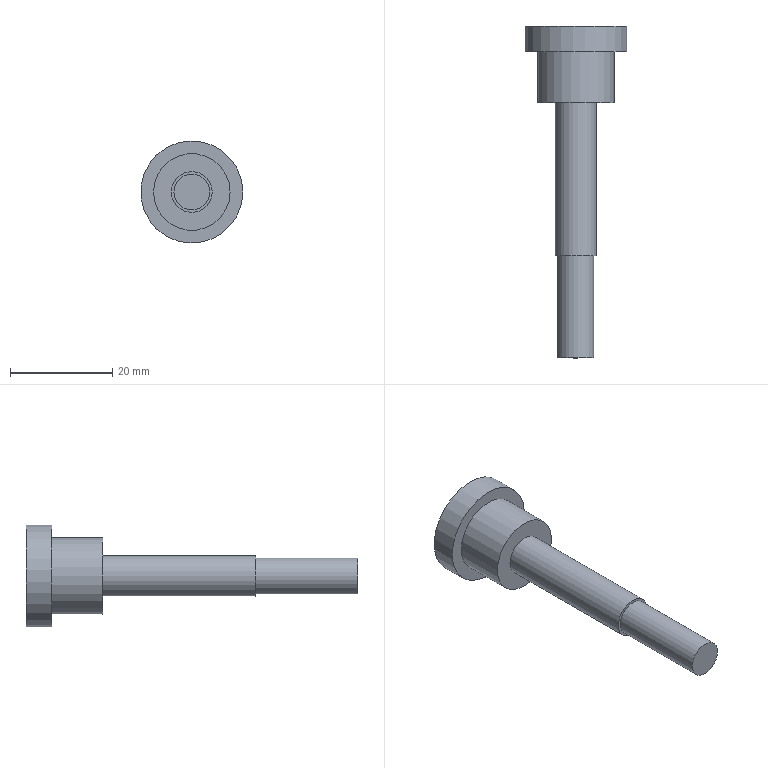Component | NX | HANDLE | 1 solid | 9 faces | box 20 x 65 x 20 mm | volume 5616 mm3 | plane 5 | cylinder 4 | commonest cylinder face diameters 7 x1 8 x1 15 x1 20 x1
STEP:
#1=CARTESIAN_POINT('',(0.,0.,0.));
#2=DIRECTION('',(0.,0.,1.));
#3=DIRECTION('',(1.,0.,0.));
#4=AXIS2_PLACEMENT_3D('',#1,#2,#3);
#5=CARTESIAN_POINT('',(28.011,213.604,30.));
#6=VERTEX_POINT('',#5);
#7=CARTESIAN_POINT('',(24.511,213.604,30.));
#8=DIRECTION('',(0.,1.,0.));
#9=DIRECTION('',(1.,0.,0.));
#10=AXIS2_PLACEMENT_3D('',#7,#8,#9);
#11=CIRCLE('',#10,3.5);
#12=CARTESIAN_POINT('',(24.511,213.604,30.));
#13=DIRECTION('',(0.,-1.,0.));
#14=DIRECTION('',(-1.,0.,0.));
#15=AXIS2_PLACEMENT_3D('',#12,#13,#14);
#16=CYLINDRICAL_SURFACE('',#15,3.5);
#17=CARTESIAN_POINT('',(9.425,0.));
#18=DIRECTION('',(-1.,0.));
#19=VECTOR('',#18,1.);
#20=LINE('',#17,#19);
#21=(GEOMETRIC_REPRESENTATION_CONTEXT(2)PARAMETRIC_REPRESENTATION_CONTEXT()REPRESENTATION_CONTEXT('',''));
#22=DEFINITIONAL_REPRESENTATION('',(#20),#21);
#23=PCURVE('',#16,#22);
#24=CARTESIAN_POINT('',(24.511,213.604,30.));
#25=DIRECTION('',(0.,1.,0.));
#26=DIRECTION('',(1.,0.,0.));
#27=AXIS2_PLACEMENT_3D('',#24,#25,#26);
#28=PLANE('',#27);
#29=CARTESIAN_POINT('',(0.,0.));
#30=DIRECTION('',(1.,0.));
#31=AXIS2_PLACEMENT_2D('',#29,#30);
#32=CIRCLE('',#31,3.5);
#33=(GEOMETRIC_REPRESENTATION_CONTEXT(2)PARAMETRIC_REPRESENTATION_CONTEXT()REPRESENTATION_CONTEXT('',''));
#34=DEFINITIONAL_REPRESENTATION('',(#32),#33);
#35=PCURVE('',#28,#34);
#36=SURFACE_CURVE('',#11,(#23,#35),.PCURVE_S1.);
#37=EDGE_CURVE('',#6,#6,#36,.T.);
#38=ORIENTED_EDGE('',*,*,#37,.F.);
#39=CARTESIAN_POINT('',(28.011,193.604,30.));
#40=VERTEX_POINT('',#39);
#41=CARTESIAN_POINT('',(28.011,213.604,30.));
#42=CARTESIAN_POINT('',(28.011,193.604,30.));
#43=B_SPLINE_CURVE_WITH_KNOTS('',1,(#41,#42),.UNSPECIFIED.,.F.,.F.,(2,2),(0.,20.),.PIECEWISE_BEZIER_KNOTS.);
#44=CARTESIAN_POINT('',(9.425,0.));
#45=DIRECTION('',(0.,1.));
#46=VECTOR('',#45,1.);
#47=LINE('',#44,#46);
#48=(GEOMETRIC_REPRESENTATION_CONTEXT(2)PARAMETRIC_REPRESENTATION_CONTEXT()REPRESENTATION_CONTEXT('',''));
#49=DEFINITIONAL_REPRESENTATION('',(#47),#48);
#50=PCURVE('',#16,#49);
#51=CARTESIAN_POINT('',(3.142,0.));
#52=DIRECTION('',(0.,1.));
#53=VECTOR('',#52,1.);
#54=LINE('',#51,#53);
#55=(GEOMETRIC_REPRESENTATION_CONTEXT(2)PARAMETRIC_REPRESENTATION_CONTEXT()REPRESENTATION_CONTEXT('',''));
#56=DEFINITIONAL_REPRESENTATION('',(#54),#55);
#57=PCURVE('',#16,#56);
#58=SEAM_CURVE('',#43,(#50,#57),.PCURVE_S1.);
#59=EDGE_CURVE('',#6,#40,#58,.T.);
#60=ORIENTED_EDGE('',*,*,#59,.T.);
#61=CARTESIAN_POINT('',(24.511,193.604,30.));
#62=DIRECTION('',(0.,1.,0.));
#63=DIRECTION('',(1.,0.,0.));
#64=AXIS2_PLACEMENT_3D('',#61,#62,#63);
#65=CIRCLE('',#64,3.5);
#66=CARTESIAN_POINT('',(9.425,20.));
#67=DIRECTION('',(-1.,0.));
#68=VECTOR('',#67,1.);
#69=LINE('',#66,#68);
#70=(GEOMETRIC_REPRESENTATION_CONTEXT(2)PARAMETRIC_REPRESENTATION_CONTEXT()REPRESENTATION_CONTEXT('',''));
#71=DEFINITIONAL_REPRESENTATION('',(#69),#70);
#72=PCURVE('',#16,#71);
#73=CARTESIAN_POINT('',(24.511,193.604,30.));
#74=DIRECTION('',(0.,1.,0.));
#75=DIRECTION('',(1.,0.,0.));
#76=AXIS2_PLACEMENT_3D('',#73,#74,#75);
#77=PLANE('',#76);
#78=CARTESIAN_POINT('',(0.,0.));
#79=DIRECTION('',(1.,0.));
#80=AXIS2_PLACEMENT_2D('',#78,#79);
#81=CIRCLE('',#80,3.5);
#82=(GEOMETRIC_REPRESENTATION_CONTEXT(2)PARAMETRIC_REPRESENTATION_CONTEXT()REPRESENTATION_CONTEXT('',''));
#83=DEFINITIONAL_REPRESENTATION('',(#81),#82);
#84=PCURVE('',#77,#83);
#85=SURFACE_CURVE('',#65,(#72,#84),.PCURVE_S1.);
#86=EDGE_CURVE('',#40,#40,#85,.T.);
#87=ORIENTED_EDGE('',*,*,#86,.T.);
#88=ORIENTED_EDGE('',*,*,#59,.F.);
#89=EDGE_LOOP('',(#38,#60,#87,#88));
#90=FACE_BOUND('',#89,.T.);
#91=ADVANCED_FACE('',(#90),#16,.T.);
#92=ORIENTED_EDGE('',*,*,#86,.F.);
#93=EDGE_LOOP('',(#92));
#94=FACE_BOUND('',#93,.T.);
#95=ADVANCED_FACE('',(#94),#77,.F.);
#96=CARTESIAN_POINT('',(28.511,243.604,30.));
#97=VERTEX_POINT('',#96);
#98=CARTESIAN_POINT('',(24.511,243.604,30.));
#99=DIRECTION('',(0.,1.,0.));
#100=DIRECTION('',(1.,0.,0.));
#101=AXIS2_PLACEMENT_3D('',#98,#99,#100);
#102=CIRCLE('',#101,4.);
#103=CARTESIAN_POINT('',(24.511,243.604,30.));
#104=DIRECTION('',(0.,-1.,0.));
#105=DIRECTION('',(-1.,0.,0.));
#106=AXIS2_PLACEMENT_3D('',#103,#104,#105);
#107=CYLINDRICAL_SURFACE('',#106,4.);
#108=CARTESIAN_POINT('',(9.425,0.));
#109=DIRECTION('',(-1.,0.));
#110=VECTOR('',#109,1.);
#111=LINE('',#108,#110);
#112=(GEOMETRIC_REPRESENTATION_CONTEXT(2)PARAMETRIC_REPRESENTATION_CONTEXT()REPRESENTATION_CONTEXT('',''));
#113=DEFINITIONAL_REPRESENTATION('',(#111),#112);
#114=PCURVE('',#107,#113);
#115=CARTESIAN_POINT('',(24.511,243.604,30.));
#116=DIRECTION('',(0.,1.,0.));
#117=DIRECTION('',(1.,0.,0.));
#118=AXIS2_PLACEMENT_3D('',#115,#116,#117);
#119=PLANE('',#118);
#120=CARTESIAN_POINT('',(0.,0.));
#121=DIRECTION('',(1.,0.));
#122=AXIS2_PLACEMENT_2D('',#120,#121);
#123=CIRCLE('',#122,4.);
#124=(GEOMETRIC_REPRESENTATION_CONTEXT(2)PARAMETRIC_REPRESENTATION_CONTEXT()REPRESENTATION_CONTEXT('',''));
#125=DEFINITIONAL_REPRESENTATION('',(#123),#124);
#126=PCURVE('',#119,#125);
#127=SURFACE_CURVE('',#102,(#114,#126),.PCURVE_S1.);
#128=EDGE_CURVE('',#97,#97,#127,.T.);
#129=ORIENTED_EDGE('',*,*,#128,.F.);
#130=CARTESIAN_POINT('',(28.511,213.604,30.));
#131=VERTEX_POINT('',#130);
#132=CARTESIAN_POINT('',(28.511,243.604,30.));
#133=CARTESIAN_POINT('',(28.511,213.604,30.));
#134=B_SPLINE_CURVE_WITH_KNOTS('',1,(#132,#133),.UNSPECIFIED.,.F.,.F.,(2,2),(0.,30.),.PIECEWISE_BEZIER_KNOTS.);
#135=CARTESIAN_POINT('',(9.425,0.));
#136=DIRECTION('',(0.,1.));
#137=VECTOR('',#136,1.);
#138=LINE('',#135,#137);
#139=(GEOMETRIC_REPRESENTATION_CONTEXT(2)PARAMETRIC_REPRESENTATION_CONTEXT()REPRESENTATION_CONTEXT('',''));
#140=DEFINITIONAL_REPRESENTATION('',(#138),#139);
#141=PCURVE('',#107,#140);
#142=CARTESIAN_POINT('',(3.142,0.));
#143=DIRECTION('',(0.,1.));
#144=VECTOR('',#143,1.);
#145=LINE('',#142,#144);
#146=(GEOMETRIC_REPRESENTATION_CONTEXT(2)PARAMETRIC_REPRESENTATION_CONTEXT()REPRESENTATION_CONTEXT('',''));
#147=DEFINITIONAL_REPRESENTATION('',(#145),#146);
#148=PCURVE('',#107,#147);
#149=SEAM_CURVE('',#134,(#141,#148),.PCURVE_S1.);
#150=EDGE_CURVE('',#97,#131,#149,.T.);
#151=ORIENTED_EDGE('',*,*,#150,.T.);
#152=CARTESIAN_POINT('',(24.511,213.604,30.));
#153=DIRECTION('',(0.,1.,0.));
#154=DIRECTION('',(1.,0.,0.));
#155=AXIS2_PLACEMENT_3D('',#152,#153,#154);
#156=CIRCLE('',#155,4.);
#157=CARTESIAN_POINT('',(9.425,30.));
#158=DIRECTION('',(-1.,0.));
#159=VECTOR('',#158,1.);
#160=LINE('',#157,#159);
#161=(GEOMETRIC_REPRESENTATION_CONTEXT(2)PARAMETRIC_REPRESENTATION_CONTEXT()REPRESENTATION_CONTEXT('',''));
#162=DEFINITIONAL_REPRESENTATION('',(#160),#161);
#163=PCURVE('',#107,#162);
#164=CARTESIAN_POINT('',(0.,0.));
#165=DIRECTION('',(1.,0.));
#166=AXIS2_PLACEMENT_2D('',#164,#165);
#167=CIRCLE('',#166,4.);
#168=(GEOMETRIC_REPRESENTATION_CONTEXT(2)PARAMETRIC_REPRESENTATION_CONTEXT()REPRESENTATION_CONTEXT('',''));
#169=DEFINITIONAL_REPRESENTATION('',(#167),#168);
#170=PCURVE('',#28,#169);
#171=SURFACE_CURVE('',#156,(#163,#170),.PCURVE_S1.);
#172=EDGE_CURVE('',#131,#131,#171,.T.);
#173=ORIENTED_EDGE('',*,*,#172,.T.);
#174=ORIENTED_EDGE('',*,*,#150,.F.);
#175=EDGE_LOOP('',(#129,#151,#173,#174));
#176=FACE_BOUND('',#175,.T.);
#177=ADVANCED_FACE('',(#176),#107,.T.);
#178=ORIENTED_EDGE('',*,*,#37,.T.);
#179=EDGE_LOOP('',(#178));
#180=FACE_BOUND('',#179,.T.);
#181=ORIENTED_EDGE('',*,*,#172,.F.);
#182=EDGE_LOOP('',(#181));
#183=FACE_BOUND('',#182,.T.);
#184=ADVANCED_FACE('',(#180,#183),#28,.F.);
#185=CARTESIAN_POINT('',(32.011,253.604,30.));
#186=VERTEX_POINT('',#185);
#187=CARTESIAN_POINT('',(24.511,253.604,30.));
#188=DIRECTION('',(0.,1.,0.));
#189=DIRECTION('',(1.,0.,0.));
#190=AXIS2_PLACEMENT_3D('',#187,#188,#189);
#191=CIRCLE('',#190,7.5);
#192=CARTESIAN_POINT('',(24.511,253.604,30.));
#193=DIRECTION('',(0.,-1.,0.));
#194=DIRECTION('',(-1.,0.,0.));
#195=AXIS2_PLACEMENT_3D('',#192,#193,#194);
#196=CYLINDRICAL_SURFACE('',#195,7.5);
#197=CARTESIAN_POINT('',(9.425,0.));
#198=DIRECTION('',(-1.,0.));
#199=VECTOR('',#198,1.);
#200=LINE('',#197,#199);
#201=(GEOMETRIC_REPRESENTATION_CONTEXT(2)PARAMETRIC_REPRESENTATION_CONTEXT()REPRESENTATION_CONTEXT('',''));
#202=DEFINITIONAL_REPRESENTATION('',(#200),#201);
#203=PCURVE('',#196,#202);
#204=CARTESIAN_POINT('',(24.511,253.604,30.));
#205=DIRECTION('',(0.,1.,0.));
#206=DIRECTION('',(1.,0.,0.));
#207=AXIS2_PLACEMENT_3D('',#204,#205,#206);
#208=PLANE('',#207);
#209=CARTESIAN_POINT('',(0.,0.));
#210=DIRECTION('',(1.,0.));
#211=AXIS2_PLACEMENT_2D('',#209,#210);
#212=CIRCLE('',#211,7.5);
#213=(GEOMETRIC_REPRESENTATION_CONTEXT(2)PARAMETRIC_REPRESENTATION_CONTEXT()REPRESENTATION_CONTEXT('',''));
#214=DEFINITIONAL_REPRESENTATION('',(#212),#213);
#215=PCURVE('',#208,#214);
#216=SURFACE_CURVE('',#191,(#203,#215),.PCURVE_S1.);
#217=EDGE_CURVE('',#186,#186,#216,.T.);
#218=ORIENTED_EDGE('',*,*,#217,.F.);
#219=CARTESIAN_POINT('',(32.011,243.604,30.));
#220=VERTEX_POINT('',#219);
#221=CARTESIAN_POINT('',(32.011,253.604,30.));
#222=CARTESIAN_POINT('',(32.011,243.604,30.));
#223=B_SPLINE_CURVE_WITH_KNOTS('',1,(#221,#222),.UNSPECIFIED.,.F.,.F.,(2,2),(0.,10.),.PIECEWISE_BEZIER_KNOTS.);
#224=CARTESIAN_POINT('',(9.425,0.));
#225=DIRECTION('',(0.,1.));
#226=VECTOR('',#225,1.);
#227=LINE('',#224,#226);
#228=(GEOMETRIC_REPRESENTATION_CONTEXT(2)PARAMETRIC_REPRESENTATION_CONTEXT()REPRESENTATION_CONTEXT('',''));
#229=DEFINITIONAL_REPRESENTATION('',(#227),#228);
#230=PCURVE('',#196,#229);
#231=CARTESIAN_POINT('',(3.142,0.));
#232=DIRECTION('',(0.,1.));
#233=VECTOR('',#232,1.);
#234=LINE('',#231,#233);
#235=(GEOMETRIC_REPRESENTATION_CONTEXT(2)PARAMETRIC_REPRESENTATION_CONTEXT()REPRESENTATION_CONTEXT('',''));
#236=DEFINITIONAL_REPRESENTATION('',(#234),#235);
#237=PCURVE('',#196,#236);
#238=SEAM_CURVE('',#223,(#230,#237),.PCURVE_S1.);
#239=EDGE_CURVE('',#186,#220,#238,.T.);
#240=ORIENTED_EDGE('',*,*,#239,.T.);
#241=CARTESIAN_POINT('',(24.511,243.604,30.));
#242=DIRECTION('',(0.,1.,0.));
#243=DIRECTION('',(1.,0.,0.));
#244=AXIS2_PLACEMENT_3D('',#241,#242,#243);
#245=CIRCLE('',#244,7.5);
#246=CARTESIAN_POINT('',(9.425,10.));
#247=DIRECTION('',(-1.,0.));
#248=VECTOR('',#247,1.);
#249=LINE('',#246,#248);
#250=(GEOMETRIC_REPRESENTATION_CONTEXT(2)PARAMETRIC_REPRESENTATION_CONTEXT()REPRESENTATION_CONTEXT('',''));
#251=DEFINITIONAL_REPRESENTATION('',(#249),#250);
#252=PCURVE('',#196,#251);
#253=CARTESIAN_POINT('',(0.,0.));
#254=DIRECTION('',(1.,0.));
#255=AXIS2_PLACEMENT_2D('',#253,#254);
#256=CIRCLE('',#255,7.5);
#257=(GEOMETRIC_REPRESENTATION_CONTEXT(2)PARAMETRIC_REPRESENTATION_CONTEXT()REPRESENTATION_CONTEXT('',''));
#258=DEFINITIONAL_REPRESENTATION('',(#256),#257);
#259=PCURVE('',#119,#258);
#260=SURFACE_CURVE('',#245,(#252,#259),.PCURVE_S1.);
#261=EDGE_CURVE('',#220,#220,#260,.T.);
#262=ORIENTED_EDGE('',*,*,#261,.T.);
#263=ORIENTED_EDGE('',*,*,#239,.F.);
#264=EDGE_LOOP('',(#218,#240,#262,#263));
#265=FACE_BOUND('',#264,.T.);
#266=ADVANCED_FACE('',(#265),#196,.T.);
#267=ORIENTED_EDGE('',*,*,#128,.T.);
#268=EDGE_LOOP('',(#267));
#269=FACE_BOUND('',#268,.T.);
#270=ORIENTED_EDGE('',*,*,#261,.F.);
#271=EDGE_LOOP('',(#270));
#272=FACE_BOUND('',#271,.T.);
#273=ADVANCED_FACE('',(#269,#272),#119,.F.);
#274=CARTESIAN_POINT('',(34.511,258.604,30.));
#275=VERTEX_POINT('',#274);
#276=CARTESIAN_POINT('',(24.511,258.604,30.));
#277=DIRECTION('',(0.,1.,0.));
#278=DIRECTION('',(1.,0.,0.));
#279=AXIS2_PLACEMENT_3D('',#276,#277,#278);
#280=CIRCLE('',#279,10.);
#281=CARTESIAN_POINT('',(24.511,258.604,30.));
#282=DIRECTION('',(0.,-1.,0.));
#283=DIRECTION('',(-1.,0.,0.));
#284=AXIS2_PLACEMENT_3D('',#281,#282,#283);
#285=CYLINDRICAL_SURFACE('',#284,10.);
#286=CARTESIAN_POINT('',(9.425,0.));
#287=DIRECTION('',(-1.,0.));
#288=VECTOR('',#287,1.);
#289=LINE('',#286,#288);
#290=(GEOMETRIC_REPRESENTATION_CONTEXT(2)PARAMETRIC_REPRESENTATION_CONTEXT()REPRESENTATION_CONTEXT('',''));
#291=DEFINITIONAL_REPRESENTATION('',(#289),#290);
#292=PCURVE('',#285,#291);
#293=CARTESIAN_POINT('',(24.511,258.604,30.));
#294=DIRECTION('',(0.,1.,0.));
#295=DIRECTION('',(1.,0.,0.));
#296=AXIS2_PLACEMENT_3D('',#293,#294,#295);
#297=PLANE('',#296);
#298=CARTESIAN_POINT('',(0.,0.));
#299=DIRECTION('',(1.,0.));
#300=AXIS2_PLACEMENT_2D('',#298,#299);
#301=CIRCLE('',#300,10.);
#302=(GEOMETRIC_REPRESENTATION_CONTEXT(2)PARAMETRIC_REPRESENTATION_CONTEXT()REPRESENTATION_CONTEXT('',''));
#303=DEFINITIONAL_REPRESENTATION('',(#301),#302);
#304=PCURVE('',#297,#303);
#305=SURFACE_CURVE('',#280,(#292,#304),.PCURVE_S1.);
#306=EDGE_CURVE('',#275,#275,#305,.T.);
#307=ORIENTED_EDGE('',*,*,#306,.F.);
#308=CARTESIAN_POINT('',(34.511,253.604,30.));
#309=VERTEX_POINT('',#308);
#310=CARTESIAN_POINT('',(34.511,258.604,30.));
#311=CARTESIAN_POINT('',(34.511,253.604,30.));
#312=B_SPLINE_CURVE_WITH_KNOTS('',1,(#310,#311),.UNSPECIFIED.,.F.,.F.,(2,2),(0.,5.),.PIECEWISE_BEZIER_KNOTS.);
#313=CARTESIAN_POINT('',(9.425,0.));
#314=DIRECTION('',(0.,1.));
#315=VECTOR('',#314,1.);
#316=LINE('',#313,#315);
#317=(GEOMETRIC_REPRESENTATION_CONTEXT(2)PARAMETRIC_REPRESENTATION_CONTEXT()REPRESENTATION_CONTEXT('',''));
#318=DEFINITIONAL_REPRESENTATION('',(#316),#317);
#319=PCURVE('',#285,#318);
#320=CARTESIAN_POINT('',(3.142,0.));
#321=DIRECTION('',(0.,1.));
#322=VECTOR('',#321,1.);
#323=LINE('',#320,#322);
#324=(GEOMETRIC_REPRESENTATION_CONTEXT(2)PARAMETRIC_REPRESENTATION_CONTEXT()REPRESENTATION_CONTEXT('',''));
#325=DEFINITIONAL_REPRESENTATION('',(#323),#324);
#326=PCURVE('',#285,#325);
#327=SEAM_CURVE('',#312,(#319,#326),.PCURVE_S1.);
#328=EDGE_CURVE('',#275,#309,#327,.T.);
#329=ORIENTED_EDGE('',*,*,#328,.T.);
#330=CARTESIAN_POINT('',(24.511,253.604,30.));
#331=DIRECTION('',(0.,1.,0.));
#332=DIRECTION('',(1.,0.,0.));
#333=AXIS2_PLACEMENT_3D('',#330,#331,#332);
#334=CIRCLE('',#333,10.);
#335=CARTESIAN_POINT('',(9.425,5.));
#336=DIRECTION('',(-1.,0.));
#337=VECTOR('',#336,1.);
#338=LINE('',#335,#337);
#339=(GEOMETRIC_REPRESENTATION_CONTEXT(2)PARAMETRIC_REPRESENTATION_CONTEXT()REPRESENTATION_CONTEXT('',''));
#340=DEFINITIONAL_REPRESENTATION('',(#338),#339);
#341=PCURVE('',#285,#340);
#342=CARTESIAN_POINT('',(0.,0.));
#343=DIRECTION('',(1.,0.));
#344=AXIS2_PLACEMENT_2D('',#342,#343);
#345=CIRCLE('',#344,10.);
#346=(GEOMETRIC_REPRESENTATION_CONTEXT(2)PARAMETRIC_REPRESENTATION_CONTEXT()REPRESENTATION_CONTEXT('',''));
#347=DEFINITIONAL_REPRESENTATION('',(#345),#346);
#348=PCURVE('',#208,#347);
#349=SURFACE_CURVE('',#334,(#341,#348),.PCURVE_S1.);
#350=EDGE_CURVE('',#309,#309,#349,.T.);
#351=ORIENTED_EDGE('',*,*,#350,.T.);
#352=ORIENTED_EDGE('',*,*,#328,.F.);
#353=EDGE_LOOP('',(#307,#329,#351,#352));
#354=FACE_BOUND('',#353,.T.);
#355=ADVANCED_FACE('',(#354),#285,.T.);
#356=ORIENTED_EDGE('',*,*,#306,.T.);
#357=EDGE_LOOP('',(#356));
#358=FACE_BOUND('',#357,.T.);
#359=ADVANCED_FACE('',(#358),#297,.T.);
#360=ORIENTED_EDGE('',*,*,#217,.T.);
#361=EDGE_LOOP('',(#360));
#362=FACE_BOUND('',#361,.T.);
#363=ORIENTED_EDGE('',*,*,#350,.F.);
#364=EDGE_LOOP('',(#363));
#365=FACE_BOUND('',#364,.T.);
#366=ADVANCED_FACE('',(#362,#365),#208,.F.);
#367=CLOSED_SHELL('',(#91,#95,#177,#184,#266,#273,#355,#359,#366));
#368=MANIFOLD_SOLID_BREP('',#367);
#369=(LENGTH_UNIT()NAMED_UNIT(*)SI_UNIT(.MILLI.,.METRE.));
#370=UNCERTAINTY_MEASURE_WITH_UNIT(LENGTH_MEASURE(0.00001),#369,'','');
#371=(NAMED_UNIT(*)PLANE_ANGLE_UNIT()SI_UNIT($,.RADIAN.));
#372=(NAMED_UNIT(*)SI_UNIT($,.STERADIAN.)SOLID_ANGLE_UNIT());
#373=(GEOMETRIC_REPRESENTATION_CONTEXT(3)GLOBAL_UNCERTAINTY_ASSIGNED_CONTEXT((#370))GLOBAL_UNIT_ASSIGNED_CONTEXT((#369,#371,#372))REPRESENTATION_CONTEXT('',''));
#374=ADVANCED_BREP_SHAPE_REPRESENTATION('',(#4,#368),#373);